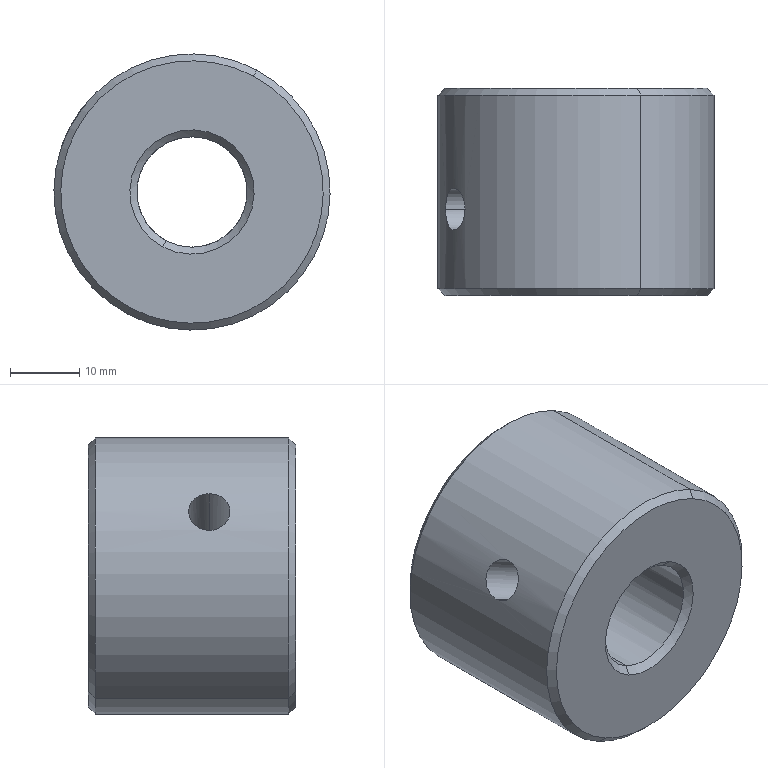Component | SolidWorks | TopMaterialTray-4 | 1 solid | 16 faces | box 40 x 30 x 40 mm | volume 31150 mm3 | cone 8 | cylinder 6 | plane 2 | commonest cylinder face diameters 6 x2 40 x2 16 x2
STEP:
#1=CARTESIAN_POINT('',(5.47,-4.508,-5.24));
#2=VERTEX_POINT('',#1);
#3=CARTESIAN_POINT('',(5.359,-4.508,-5.449));
#4=VERTEX_POINT('',#3);
#5=CARTESIAN_POINT('',(5.47,-4.508,-5.24));
#6=CARTESIAN_POINT('',(5.47,-4.516,-5.24));
#7=CARTESIAN_POINT('',(5.469,-4.523,-5.241));
#8=CARTESIAN_POINT('',(5.467,-4.539,-5.243));
#9=CARTESIAN_POINT('',(5.466,-4.546,-5.245));
#10=CARTESIAN_POINT('',(5.463,-4.56,-5.25));
#11=CARTESIAN_POINT('',(5.46,-4.567,-5.253));
#12=CARTESIAN_POINT('',(5.455,-4.58,-5.26));
#13=CARTESIAN_POINT('',(5.453,-4.586,-5.264));
#14=CARTESIAN_POINT('',(5.446,-4.597,-5.273));
#15=CARTESIAN_POINT('',(5.443,-4.602,-5.278));
#16=CARTESIAN_POINT('',(5.436,-4.61,-5.289));
#17=CARTESIAN_POINT('',(5.433,-4.614,-5.295));
#18=CARTESIAN_POINT('',(5.425,-4.62,-5.307));
#19=CARTESIAN_POINT('',(5.421,-4.622,-5.313));
#20=CARTESIAN_POINT('',(5.414,-4.625,-5.326));
#21=CARTESIAN_POINT('',(5.41,-4.626,-5.333));
#22=CARTESIAN_POINT('',(5.403,-4.626,-5.347));
#23=CARTESIAN_POINT('',(5.399,-4.625,-5.354));
#24=CARTESIAN_POINT('',(5.393,-4.622,-5.367));
#25=CARTESIAN_POINT('',(5.389,-4.62,-5.374));
#26=CARTESIAN_POINT('',(5.384,-4.614,-5.387));
#27=CARTESIAN_POINT('',(5.381,-4.61,-5.393));
#28=CARTESIAN_POINT('',(5.376,-4.602,-5.405));
#29=CARTESIAN_POINT('',(5.373,-4.597,-5.411));
#30=CARTESIAN_POINT('',(5.369,-4.586,-5.421));
#31=CARTESIAN_POINT('',(5.368,-4.58,-5.426));
#32=CARTESIAN_POINT('',(5.364,-4.567,-5.434));
#33=CARTESIAN_POINT('',(5.363,-4.56,-5.437));
#34=CARTESIAN_POINT('',(5.361,-4.546,-5.443));
#35=CARTESIAN_POINT('',(5.36,-4.539,-5.445));
#36=CARTESIAN_POINT('',(5.359,-4.523,-5.448));
#37=CARTESIAN_POINT('',(5.359,-4.516,-5.449));
#38=CARTESIAN_POINT('',(5.359,-4.508,-5.449));
#39=B_SPLINE_CURVE_WITH_KNOTS('',3,(#5,#6,#7,#8,#9,#10,#11,#12,#13,#14,#15,#16,#17,#18,#19,#20,#21,#22,#23,#24,#25,#26,#27,#28,#29,#30,#31,#32,#33,#34,#35,#36,#37,#38),.UNSPECIFIED.,.F.,.F.,(4,2,2,2,2,2,2,2,2,2,2,2,2,2,2,2,4),(0.009393,0.00998,0.01057,0.01115,0.01174,0.01233,0.01291,0.0135,0.01409,0.01467,0.01526,0.01585,0.01644,0.01702,0.01761,0.0182,0.01878),.UNSPECIFIED.);
#40=EDGE_CURVE('',#2,#4,#39,.T.);
#41=ORIENTED_EDGE('',*,*,#40,.F.);
#42=CARTESIAN_POINT('',(5.9,-4.508,-5.468));
#43=VERTEX_POINT('',#42);
#44=CARTESIAN_POINT('',(6.018,-4.508,-5.531));
#45=DIRECTION('',(0.8837,-0.,-0.468));
#46=VECTOR('',#45,39.37);
#47=LINE('',#44,#46);
#48=EDGE_CURVE('',#2,#43,#47,.T.);
#49=ORIENTED_EDGE('',*,*,#48,.T.);
#50=CARTESIAN_POINT('',(5.789,-4.508,-5.676));
#51=VERTEX_POINT('',#50);
#52=CARTESIAN_POINT('',(5.9,-4.508,-5.468));
#53=CARTESIAN_POINT('',(5.9,-4.516,-5.468));
#54=CARTESIAN_POINT('',(5.899,-4.523,-5.468));
#55=CARTESIAN_POINT('',(5.896,-4.539,-5.47));
#56=CARTESIAN_POINT('',(5.895,-4.546,-5.472));
#57=CARTESIAN_POINT('',(5.89,-4.56,-5.476));
#58=CARTESIAN_POINT('',(5.887,-4.567,-5.479));
#59=CARTESIAN_POINT('',(5.881,-4.58,-5.485));
#60=CARTESIAN_POINT('',(5.877,-4.586,-5.489));
#61=CARTESIAN_POINT('',(5.869,-4.597,-5.497));
#62=CARTESIAN_POINT('',(5.865,-4.602,-5.501));
#63=CARTESIAN_POINT('',(5.857,-4.61,-5.511));
#64=CARTESIAN_POINT('',(5.852,-4.614,-5.517));
#65=CARTESIAN_POINT('',(5.844,-4.62,-5.529));
#66=CARTESIAN_POINT('',(5.84,-4.622,-5.535));
#67=CARTESIAN_POINT('',(5.832,-4.625,-5.548));
#68=CARTESIAN_POINT('',(5.828,-4.626,-5.554));
#69=CARTESIAN_POINT('',(5.82,-4.626,-5.568));
#70=CARTESIAN_POINT('',(5.817,-4.625,-5.575));
#71=CARTESIAN_POINT('',(5.811,-4.622,-5.589));
#72=CARTESIAN_POINT('',(5.808,-4.62,-5.596));
#73=CARTESIAN_POINT('',(5.803,-4.614,-5.61));
#74=CARTESIAN_POINT('',(5.801,-4.61,-5.616));
#75=CARTESIAN_POINT('',(5.798,-4.602,-5.629));
#76=CARTESIAN_POINT('',(5.796,-4.597,-5.635));
#77=CARTESIAN_POINT('',(5.794,-4.586,-5.646));
#78=CARTESIAN_POINT('',(5.793,-4.58,-5.651));
#79=CARTESIAN_POINT('',(5.791,-4.567,-5.66));
#80=CARTESIAN_POINT('',(5.791,-4.56,-5.664));
#81=CARTESIAN_POINT('',(5.79,-4.546,-5.67));
#82=CARTESIAN_POINT('',(5.79,-4.539,-5.672));
#83=CARTESIAN_POINT('',(5.789,-4.523,-5.676));
#84=CARTESIAN_POINT('',(5.789,-4.516,-5.676));
#85=CARTESIAN_POINT('',(5.789,-4.508,-5.676));
#86=B_SPLINE_CURVE_WITH_KNOTS('',3,(#52,#53,#54,#55,#56,#57,#58,#59,#60,#61,#62,#63,#64,#65,#66,#67,#68,#69,#70,#71,#72,#73,#74,#75,#76,#77,#78,#79,#80,#81,#82,#83,#84,#85),.UNSPECIFIED.,.F.,.F.,(4,2,2,2,2,2,2,2,2,2,2,2,2,2,2,2,4),(0.009466,0.01006,0.01065,0.01124,0.01183,0.01242,0.01302,0.01361,0.0142,0.01479,0.01538,0.01597,0.01656,0.01716,0.01775,0.01834,0.01893),.UNSPECIFIED.);
#87=EDGE_CURVE('',#43,#51,#86,.T.);
#88=ORIENTED_EDGE('',*,*,#87,.T.);
#89=CARTESIAN_POINT('',(5.908,-4.508,-5.739));
#90=DIRECTION('',(0.8837,-0.,-0.468));
#91=VECTOR('',#90,39.37);
#92=LINE('',#89,#91);
#93=EDGE_CURVE('',#4,#51,#92,.T.);
#94=ORIENTED_EDGE('',*,*,#93,.F.);
#95=EDGE_LOOP('',(#41,#49,#88,#94));
#96=FACE_OUTER_BOUND('',#95,.T.);
#97=CARTESIAN_POINT('',(5.963,-4.508,-5.635));
#98=DIRECTION('',(0.8837,-0.,-0.468));
#99=DIRECTION('',(-0.468,0.,-0.8837));
#100=AXIS2_PLACEMENT_3D('',#97,#98,#99);
#101=CYLINDRICAL_SURFACE('',#100,0.1181);
#102=ADVANCED_FACE('',(#96),#101,.F.);
#103=CARTESIAN_POINT('',(5.752,-5.,-6.37));
#104=VERTEX_POINT('',#103);
#105=CARTESIAN_POINT('',(6.452,-5.,-5.048));
#106=VERTEX_POINT('',#105);
#107=CARTESIAN_POINT('',(6.102,-5.,-5.709));
#108=DIRECTION('',(0.,1.,0.));
#109=DIRECTION('',(-0.468,0.,-0.8837));
#110=AXIS2_PLACEMENT_3D('',#107,#108,#109);
#111=CIRCLE('',#110,0.748);
#112=EDGE_CURVE('',#104,#106,#111,.T.);
#113=ORIENTED_EDGE('',*,*,#112,.T.);
#114=CARTESIAN_POINT('',(6.471,-4.961,-5.013));
#115=VERTEX_POINT('',#114);
#116=CARTESIAN_POINT('',(6.471,-4.961,-5.013));
#117=DIRECTION('',(0.3309,0.7071,0.6249));
#118=VECTOR('',#117,39.37);
#119=LINE('',#116,#118);
#120=EDGE_CURVE('',#106,#115,#119,.T.);
#121=ORIENTED_EDGE('',*,*,#120,.T.);
#122=CARTESIAN_POINT('',(5.734,-4.961,-6.405));
#123=VERTEX_POINT('',#122);
#124=CARTESIAN_POINT('',(6.102,-4.961,-5.709));
#125=DIRECTION('',(0.,1.,0.));
#126=DIRECTION('',(0.468,-0.,0.8837));
#127=AXIS2_PLACEMENT_3D('',#124,#125,#126);
#128=CIRCLE('',#127,0.7874);
#129=EDGE_CURVE('',#123,#115,#128,.T.);
#130=ORIENTED_EDGE('',*,*,#129,.F.);
#131=CARTESIAN_POINT('',(5.734,-4.961,-6.405));
#132=DIRECTION('',(-0.3309,0.7071,-0.6249));
#133=VECTOR('',#132,39.37);
#134=LINE('',#131,#133);
#135=EDGE_CURVE('',#104,#123,#134,.T.);
#136=ORIENTED_EDGE('',*,*,#135,.F.);
#137=EDGE_LOOP('',(#113,#121,#130,#136));
#138=FACE_OUTER_BOUND('',#137,.T.);
#139=CARTESIAN_POINT('',(6.102,-4.961,-5.709));
#140=DIRECTION('',(0.,1.,0.));
#141=DIRECTION('',(-0.468,0.,-0.8837));
#142=AXIS2_PLACEMENT_3D('',#139,#140,#141);
#143=CONICAL_SURFACE('',#142,0.7874,0.7854);
#144=ADVANCED_FACE('',(#138),#143,.T.);
#145=CARTESIAN_POINT('',(6.452,-3.819,-5.048));
#146=VERTEX_POINT('',#145);
#147=CARTESIAN_POINT('',(5.752,-3.819,-6.37));
#148=VERTEX_POINT('',#147);
#149=CARTESIAN_POINT('',(6.102,-3.819,-5.709));
#150=DIRECTION('',(-0.,-1.,-0.));
#151=DIRECTION('',(0.468,-0.,0.8837));
#152=AXIS2_PLACEMENT_3D('',#149,#150,#151);
#153=CIRCLE('',#152,0.748);
#154=EDGE_CURVE('',#146,#148,#153,.T.);
#155=ORIENTED_EDGE('',*,*,#154,.T.);
#156=CARTESIAN_POINT('',(5.734,-3.858,-6.405));
#157=VERTEX_POINT('',#156);
#158=CARTESIAN_POINT('',(5.734,-3.858,-6.405));
#159=DIRECTION('',(-0.3309,-0.7071,-0.6249));
#160=VECTOR('',#159,39.37);
#161=LINE('',#158,#160);
#162=EDGE_CURVE('',#148,#157,#161,.T.);
#163=ORIENTED_EDGE('',*,*,#162,.T.);
#164=CARTESIAN_POINT('',(6.471,-3.858,-5.013));
#165=VERTEX_POINT('',#164);
#166=CARTESIAN_POINT('',(6.102,-3.858,-5.709));
#167=DIRECTION('',(-0.,-1.,-0.));
#168=DIRECTION('',(0.468,-0.,0.8837));
#169=AXIS2_PLACEMENT_3D('',#166,#167,#168);
#170=CIRCLE('',#169,0.7874);
#171=EDGE_CURVE('',#165,#157,#170,.T.);
#172=ORIENTED_EDGE('',*,*,#171,.F.);
#173=CARTESIAN_POINT('',(6.471,-3.858,-5.013));
#174=DIRECTION('',(0.3309,-0.7071,0.6249));
#175=VECTOR('',#174,39.37);
#176=LINE('',#173,#175);
#177=EDGE_CURVE('',#146,#165,#176,.T.);
#178=ORIENTED_EDGE('',*,*,#177,.F.);
#179=EDGE_LOOP('',(#155,#163,#172,#178));
#180=FACE_OUTER_BOUND('',#179,.T.);
#181=CARTESIAN_POINT('',(6.102,-3.858,-5.709));
#182=DIRECTION('',(-0.,-1.,-0.));
#183=DIRECTION('',(0.468,-0.,0.8837));
#184=AXIS2_PLACEMENT_3D('',#181,#182,#183);
#185=CONICAL_SURFACE('',#184,0.7874,0.7854);
#186=ADVANCED_FACE('',(#180),#185,.T.);
#187=CARTESIAN_POINT('',(5.955,-4.961,-5.987));
#188=VERTEX_POINT('',#187);
#189=CARTESIAN_POINT('',(6.25,-4.961,-5.43));
#190=VERTEX_POINT('',#189);
#191=CARTESIAN_POINT('',(6.102,-4.961,-5.709));
#192=DIRECTION('',(-0.,-1.,-0.));
#193=DIRECTION('',(0.468,0.,0.8837));
#194=AXIS2_PLACEMENT_3D('',#191,#192,#193);
#195=CIRCLE('',#194,0.315);
#196=EDGE_CURVE('',#188,#190,#195,.T.);
#197=ORIENTED_EDGE('',*,*,#196,.F.);
#198=CARTESIAN_POINT('',(5.937,-5.,-6.022));
#199=VERTEX_POINT('',#198);
#200=CARTESIAN_POINT('',(5.937,-5.,-6.022));
#201=DIRECTION('',(-0.3309,-0.7071,-0.6249));
#202=VECTOR('',#201,39.37);
#203=LINE('',#200,#202);
#204=EDGE_CURVE('',#188,#199,#203,.T.);
#205=ORIENTED_EDGE('',*,*,#204,.T.);
#206=CARTESIAN_POINT('',(6.268,-5.,-5.396));
#207=VERTEX_POINT('',#206);
#208=CARTESIAN_POINT('',(6.102,-5.,-5.709));
#209=DIRECTION('',(0.,1.,0.));
#210=DIRECTION('',(0.468,-0.,0.8837));
#211=AXIS2_PLACEMENT_3D('',#208,#209,#210);
#212=CIRCLE('',#211,0.3543);
#213=EDGE_CURVE('',#207,#199,#212,.T.);
#214=ORIENTED_EDGE('',*,*,#213,.F.);
#215=CARTESIAN_POINT('',(6.268,-5.,-5.396));
#216=DIRECTION('',(0.3309,-0.7071,0.6249));
#217=VECTOR('',#216,39.37);
#218=LINE('',#215,#217);
#219=EDGE_CURVE('',#190,#207,#218,.T.);
#220=ORIENTED_EDGE('',*,*,#219,.F.);
#221=EDGE_LOOP('',(#197,#205,#214,#220));
#222=FACE_OUTER_BOUND('',#221,.T.);
#223=CARTESIAN_POINT('',(6.102,-5.,-5.709));
#224=DIRECTION('',(-0.,-1.,-0.));
#225=DIRECTION('',(0.468,-0.,0.8837));
#226=AXIS2_PLACEMENT_3D('',#223,#224,#225);
#227=CONICAL_SURFACE('',#226,0.3543,0.7854);
#228=ADVANCED_FACE('',(#222),#227,.F.);
#229=CARTESIAN_POINT('',(6.25,-3.858,-5.43));
#230=VERTEX_POINT('',#229);
#231=CARTESIAN_POINT('',(5.824,-3.858,-5.561));
#232=VERTEX_POINT('',#231);
#233=CARTESIAN_POINT('',(6.102,-3.858,-5.709));
#234=DIRECTION('',(-0.,-1.,-0.));
#235=DIRECTION('',(-0.468,0.,-0.8837));
#236=AXIS2_PLACEMENT_3D('',#233,#234,#235);
#237=CIRCLE('',#236,0.315);
#238=EDGE_CURVE('',#230,#232,#237,.T.);
#239=ORIENTED_EDGE('',*,*,#238,.T.);
#240=CARTESIAN_POINT('',(5.789,-3.819,-5.543));
#241=VERTEX_POINT('',#240);
#242=CARTESIAN_POINT('',(5.789,-3.819,-5.543));
#243=DIRECTION('',(-0.6249,0.7071,0.3309));
#244=VECTOR('',#243,39.37);
#245=LINE('',#242,#244);
#246=EDGE_CURVE('',#232,#241,#245,.T.);
#247=ORIENTED_EDGE('',*,*,#246,.T.);
#248=CARTESIAN_POINT('',(6.415,-3.819,-5.874));
#249=VERTEX_POINT('',#248);
#250=CARTESIAN_POINT('',(6.102,-3.819,-5.709));
#251=DIRECTION('',(-0.,-1.,-0.));
#252=DIRECTION('',(0.8837,0.,-0.468));
#253=AXIS2_PLACEMENT_3D('',#250,#251,#252);
#254=CIRCLE('',#253,0.3543);
#255=EDGE_CURVE('',#249,#241,#254,.T.);
#256=ORIENTED_EDGE('',*,*,#255,.F.);
#257=CARTESIAN_POINT('',(6.381,-3.858,-5.856));
#258=VERTEX_POINT('',#257);
#259=CARTESIAN_POINT('',(6.415,-3.819,-5.874));
#260=DIRECTION('',(0.6249,0.7071,-0.3309));
#261=VECTOR('',#260,39.37);
#262=LINE('',#259,#261);
#263=EDGE_CURVE('',#258,#249,#262,.T.);
#264=ORIENTED_EDGE('',*,*,#263,.F.);
#265=CARTESIAN_POINT('',(6.102,-3.858,-5.709));
#266=DIRECTION('',(-0.,-1.,-0.));
#267=DIRECTION('',(-0.468,0.,-0.8837));
#268=AXIS2_PLACEMENT_3D('',#265,#266,#267);
#269=CIRCLE('',#268,0.315);
#270=EDGE_CURVE('',#258,#230,#269,.T.);
#271=ORIENTED_EDGE('',*,*,#270,.T.);
#272=EDGE_LOOP('',(#239,#247,#256,#264,#271));
#273=FACE_OUTER_BOUND('',#272,.T.);
#274=CARTESIAN_POINT('',(6.102,-3.819,-5.709));
#275=DIRECTION('',(0.,1.,0.));
#276=DIRECTION('',(0.8837,0.,-0.468));
#277=AXIS2_PLACEMENT_3D('',#274,#275,#276);
#278=CONICAL_SURFACE('',#277,0.3543,0.7854);
#279=ADVANCED_FACE('',(#273),#278,.F.);
#280=CARTESIAN_POINT('',(5.359,-4.508,-5.449));
#281=CARTESIAN_POINT('',(5.359,-4.5,-5.449));
#282=CARTESIAN_POINT('',(5.359,-4.492,-5.448));
#283=CARTESIAN_POINT('',(5.36,-4.477,-5.445));
#284=CARTESIAN_POINT('',(5.361,-4.47,-5.443));
#285=CARTESIAN_POINT('',(5.363,-4.455,-5.437));
#286=CARTESIAN_POINT('',(5.364,-4.449,-5.434));
#287=CARTESIAN_POINT('',(5.368,-4.436,-5.426));
#288=CARTESIAN_POINT('',(5.369,-4.43,-5.421));
#289=CARTESIAN_POINT('',(5.373,-4.419,-5.411));
#290=CARTESIAN_POINT('',(5.376,-4.414,-5.405));
#291=CARTESIAN_POINT('',(5.381,-4.405,-5.394));
#292=CARTESIAN_POINT('',(5.384,-4.402,-5.387));
#293=CARTESIAN_POINT('',(5.389,-4.396,-5.374));
#294=CARTESIAN_POINT('',(5.393,-4.394,-5.368));
#295=CARTESIAN_POINT('',(5.399,-4.391,-5.354));
#296=CARTESIAN_POINT('',(5.403,-4.39,-5.347));
#297=CARTESIAN_POINT('',(5.41,-4.39,-5.333));
#298=CARTESIAN_POINT('',(5.414,-4.391,-5.327));
#299=CARTESIAN_POINT('',(5.421,-4.394,-5.313));
#300=CARTESIAN_POINT('',(5.425,-4.396,-5.307));
#301=CARTESIAN_POINT('',(5.433,-4.402,-5.295));
#302=CARTESIAN_POINT('',(5.436,-4.405,-5.289));
#303=CARTESIAN_POINT('',(5.443,-4.414,-5.278));
#304=CARTESIAN_POINT('',(5.446,-4.419,-5.273));
#305=CARTESIAN_POINT('',(5.453,-4.43,-5.264));
#306=CARTESIAN_POINT('',(5.455,-4.436,-5.26));
#307=CARTESIAN_POINT('',(5.46,-4.449,-5.253));
#308=CARTESIAN_POINT('',(5.463,-4.456,-5.25));
#309=CARTESIAN_POINT('',(5.466,-4.47,-5.245));
#310=CARTESIAN_POINT('',(5.467,-4.477,-5.243));
#311=CARTESIAN_POINT('',(5.469,-4.492,-5.241));
#312=CARTESIAN_POINT('',(5.47,-4.5,-5.24));
#313=CARTESIAN_POINT('',(5.47,-4.508,-5.24));
#314=B_SPLINE_CURVE_WITH_KNOTS('',3,(#280,#281,#282,#283,#284,#285,#286,#287,#288,#289,#290,#291,#292,#293,#294,#295,#296,#297,#298,#299,#300,#301,#302,#303,#304,#305,#306,#307,#308,#309,#310,#311,#312,#313),.UNSPECIFIED.,.F.,.F.,(4,2,2,2,2,2,2,2,2,2,2,2,2,2,2,2,4),(0.,0.000587,0.001174,0.001761,0.002348,0.002935,0.003522,0.004109,0.004696,0.005283,0.00587,0.006457,0.007044,0.007631,0.008219,0.008806,0.009393),.UNSPECIFIED.);
#315=EDGE_CURVE('',#4,#2,#314,.T.);
#316=ORIENTED_EDGE('',*,*,#315,.T.);
#317=ORIENTED_EDGE('',*,*,#40,.T.);
#318=EDGE_LOOP('',(#316,#317));
#319=FACE_BOUND('',#318,.T.);
#320=ORIENTED_EDGE('',*,*,#171,.T.);
#321=CARTESIAN_POINT('',(5.734,-5.,-6.405));
#322=DIRECTION('',(-0.,-1.,-0.));
#323=VECTOR('',#322,39.37);
#324=LINE('',#321,#323);
#325=EDGE_CURVE('',#157,#123,#324,.T.);
#326=ORIENTED_EDGE('',*,*,#325,.T.);
#327=ORIENTED_EDGE('',*,*,#129,.T.);
#328=CARTESIAN_POINT('',(6.471,-5.,-5.013));
#329=DIRECTION('',(-0.,-1.,-0.));
#330=VECTOR('',#329,39.37);
#331=LINE('',#328,#330);
#332=EDGE_CURVE('',#165,#115,#331,.T.);
#333=ORIENTED_EDGE('',*,*,#332,.F.);
#334=EDGE_LOOP('',(#320,#326,#327,#333));
#335=FACE_OUTER_BOUND('',#334,.T.);
#336=CARTESIAN_POINT('',(6.102,-5.,-5.709));
#337=DIRECTION('',(-0.,-1.,-0.));
#338=DIRECTION('',(0.468,-0.,0.8837));
#339=AXIS2_PLACEMENT_3D('',#336,#337,#338);
#340=CYLINDRICAL_SURFACE('',#339,0.7874);
#341=ADVANCED_FACE('',(#319,#335),#340,.T.);
#342=ORIENTED_EDGE('',*,*,#196,.T.);
#343=CARTESIAN_POINT('',(6.25,-5.,-5.43));
#344=DIRECTION('',(0.,1.,0.));
#345=VECTOR('',#344,39.37);
#346=LINE('',#343,#345);
#347=EDGE_CURVE('',#190,#230,#346,.T.);
#348=ORIENTED_EDGE('',*,*,#347,.T.);
#349=ORIENTED_EDGE('',*,*,#270,.F.);
#350=CARTESIAN_POINT('',(5.955,-3.858,-5.987));
#351=VERTEX_POINT('',#350);
#352=CARTESIAN_POINT('',(6.102,-3.858,-5.709));
#353=DIRECTION('',(-0.,-1.,-0.));
#354=DIRECTION('',(-0.468,0.,-0.8837));
#355=AXIS2_PLACEMENT_3D('',#352,#353,#354);
#356=CIRCLE('',#355,0.315);
#357=EDGE_CURVE('',#351,#258,#356,.T.);
#358=ORIENTED_EDGE('',*,*,#357,.F.);
#359=CARTESIAN_POINT('',(5.955,-5.,-5.987));
#360=DIRECTION('',(0.,1.,0.));
#361=VECTOR('',#360,39.37);
#362=LINE('',#359,#361);
#363=EDGE_CURVE('',#188,#351,#362,.T.);
#364=ORIENTED_EDGE('',*,*,#363,.F.);
#365=EDGE_LOOP('',(#342,#348,#349,#358,#364));
#366=FACE_OUTER_BOUND('',#365,.T.);
#367=CARTESIAN_POINT('',(6.102,-5.,-5.709));
#368=DIRECTION('',(0.,1.,0.));
#369=DIRECTION('',(-0.468,0.,-0.8837));
#370=AXIS2_PLACEMENT_3D('',#367,#368,#369);
#371=CYLINDRICAL_SURFACE('',#370,0.315);
#372=ADVANCED_FACE('',(#366),#371,.F.);
#373=ORIENTED_EDGE('',*,*,#347,.F.);
#374=CARTESIAN_POINT('',(6.102,-4.961,-5.709));
#375=DIRECTION('',(-0.,-1.,-0.));
#376=DIRECTION('',(0.468,0.,0.8837));
#377=AXIS2_PLACEMENT_3D('',#374,#375,#376);
#378=CIRCLE('',#377,0.315);
#379=EDGE_CURVE('',#190,#188,#378,.T.);
#380=ORIENTED_EDGE('',*,*,#379,.T.);
#381=ORIENTED_EDGE('',*,*,#363,.T.);
#382=CARTESIAN_POINT('',(6.102,-3.858,-5.709));
#383=DIRECTION('',(-0.,-1.,-0.));
#384=DIRECTION('',(-0.468,0.,-0.8837));
#385=AXIS2_PLACEMENT_3D('',#382,#383,#384);
#386=CIRCLE('',#385,0.315);
#387=EDGE_CURVE('',#232,#351,#386,.T.);
#388=ORIENTED_EDGE('',*,*,#387,.F.);
#389=ORIENTED_EDGE('',*,*,#238,.F.);
#390=EDGE_LOOP('',(#373,#380,#381,#388,#389));
#391=FACE_OUTER_BOUND('',#390,.T.);
#392=CARTESIAN_POINT('',(5.789,-4.508,-5.676));
#393=CARTESIAN_POINT('',(5.789,-4.5,-5.676));
#394=CARTESIAN_POINT('',(5.789,-4.492,-5.676));
#395=CARTESIAN_POINT('',(5.79,-4.477,-5.672));
#396=CARTESIAN_POINT('',(5.79,-4.47,-5.67));
#397=CARTESIAN_POINT('',(5.791,-4.455,-5.664));
#398=CARTESIAN_POINT('',(5.791,-4.449,-5.66));
#399=CARTESIAN_POINT('',(5.793,-4.436,-5.651));
#400=CARTESIAN_POINT('',(5.794,-4.43,-5.646));
#401=CARTESIAN_POINT('',(5.797,-4.414,-5.629));
#402=CARTESIAN_POINT('',(5.801,-4.405,-5.617));
#403=CARTESIAN_POINT('',(5.808,-4.396,-5.596));
#404=CARTESIAN_POINT('',(5.811,-4.394,-5.589));
#405=CARTESIAN_POINT('',(5.817,-4.391,-5.575));
#406=CARTESIAN_POINT('',(5.82,-4.39,-5.568));
#407=CARTESIAN_POINT('',(5.828,-4.39,-5.554));
#408=CARTESIAN_POINT('',(5.832,-4.391,-5.548));
#409=CARTESIAN_POINT('',(5.84,-4.394,-5.535));
#410=CARTESIAN_POINT('',(5.844,-4.396,-5.529));
#411=CARTESIAN_POINT('',(5.853,-4.402,-5.517));
#412=CARTESIAN_POINT('',(5.857,-4.406,-5.511));
#413=CARTESIAN_POINT('',(5.865,-4.414,-5.501));
#414=CARTESIAN_POINT('',(5.869,-4.419,-5.497));
#415=CARTESIAN_POINT('',(5.877,-4.43,-5.489));
#416=CARTESIAN_POINT('',(5.881,-4.436,-5.485));
#417=CARTESIAN_POINT('',(5.887,-4.448,-5.479));
#418=CARTESIAN_POINT('',(5.89,-4.455,-5.476));
#419=CARTESIAN_POINT('',(5.895,-4.47,-5.472));
#420=CARTESIAN_POINT('',(5.896,-4.477,-5.47));
#421=CARTESIAN_POINT('',(5.899,-4.492,-5.468));
#422=CARTESIAN_POINT('',(5.9,-4.5,-5.468));
#423=CARTESIAN_POINT('',(5.9,-4.508,-5.468));
#424=B_SPLINE_CURVE_WITH_KNOTS('',3,(#392,#393,#394,#395,#396,#397,#398,#399,#400,#401,#402,#403,#404,#405,#406,#407,#408,#409,#410,#411,#412,#413,#414,#415,#416,#417,#418,#419,#420,#421,#422,#423),.UNSPECIFIED.,.F.,.F.,(4,2,2,2,2,2,2,2,2,2,2,2,2,2,2,4),(0.,0.0005916,0.001183,0.001775,0.002367,0.00355,0.004142,0.004733,0.005325,0.005916,0.006508,0.0071,0.007691,0.008283,0.008875,0.009466),.UNSPECIFIED.);
#425=EDGE_CURVE('',#51,#43,#424,.T.);
#426=ORIENTED_EDGE('',*,*,#425,.F.);
#427=ORIENTED_EDGE('',*,*,#87,.F.);
#428=EDGE_LOOP('',(#426,#427));
#429=FACE_BOUND('',#428,.T.);
#430=CARTESIAN_POINT('',(6.102,-5.,-5.709));
#431=DIRECTION('',(0.,1.,0.));
#432=DIRECTION('',(-0.468,0.,-0.8837));
#433=AXIS2_PLACEMENT_3D('',#430,#431,#432);
#434=CYLINDRICAL_SURFACE('',#433,0.315);
#435=ADVANCED_FACE('',(#391,#429),#434,.F.);
#436=ORIENTED_EDGE('',*,*,#325,.F.);
#437=CARTESIAN_POINT('',(6.102,-3.858,-5.709));
#438=DIRECTION('',(-0.,-1.,-0.));
#439=DIRECTION('',(0.468,-0.,0.8837));
#440=AXIS2_PLACEMENT_3D('',#437,#438,#439);
#441=CIRCLE('',#440,0.7874);
#442=EDGE_CURVE('',#157,#165,#441,.T.);
#443=ORIENTED_EDGE('',*,*,#442,.T.);
#444=ORIENTED_EDGE('',*,*,#332,.T.);
#445=CARTESIAN_POINT('',(6.102,-4.961,-5.709));
#446=DIRECTION('',(0.,1.,0.));
#447=DIRECTION('',(0.468,-0.,0.8837));
#448=AXIS2_PLACEMENT_3D('',#445,#446,#447);
#449=CIRCLE('',#448,0.7874);
#450=EDGE_CURVE('',#115,#123,#449,.T.);
#451=ORIENTED_EDGE('',*,*,#450,.T.);
#452=EDGE_LOOP('',(#436,#443,#444,#451));
#453=FACE_OUTER_BOUND('',#452,.T.);
#454=CARTESIAN_POINT('',(6.102,-5.,-5.709));
#455=DIRECTION('',(-0.,-1.,-0.));
#456=DIRECTION('',(0.468,-0.,0.8837));
#457=AXIS2_PLACEMENT_3D('',#454,#455,#456);
#458=CYLINDRICAL_SURFACE('',#457,0.7874);
#459=ADVANCED_FACE('',(#453),#458,.T.);
#460=ORIENTED_EDGE('',*,*,#120,.F.);
#461=CARTESIAN_POINT('',(6.102,-5.,-5.709));
#462=DIRECTION('',(0.,1.,0.));
#463=DIRECTION('',(-0.468,0.,-0.8837));
#464=AXIS2_PLACEMENT_3D('',#461,#462,#463);
#465=CIRCLE('',#464,0.748);
#466=EDGE_CURVE('',#106,#104,#465,.T.);
#467=ORIENTED_EDGE('',*,*,#466,.T.);
#468=ORIENTED_EDGE('',*,*,#135,.T.);
#469=ORIENTED_EDGE('',*,*,#450,.F.);
#470=EDGE_LOOP('',(#460,#467,#468,#469));
#471=FACE_OUTER_BOUND('',#470,.T.);
#472=CARTESIAN_POINT('',(6.102,-4.961,-5.709));
#473=DIRECTION('',(0.,1.,0.));
#474=DIRECTION('',(-0.468,0.,-0.8837));
#475=AXIS2_PLACEMENT_3D('',#472,#473,#474);
#476=CONICAL_SURFACE('',#475,0.7874,0.7854);
#477=ADVANCED_FACE('',(#471),#476,.T.);
#478=ORIENTED_EDGE('',*,*,#162,.F.);
#479=CARTESIAN_POINT('',(6.102,-3.819,-5.709));
#480=DIRECTION('',(-0.,-1.,-0.));
#481=DIRECTION('',(0.468,-0.,0.8837));
#482=AXIS2_PLACEMENT_3D('',#479,#480,#481);
#483=CIRCLE('',#482,0.748);
#484=EDGE_CURVE('',#148,#146,#483,.T.);
#485=ORIENTED_EDGE('',*,*,#484,.T.);
#486=ORIENTED_EDGE('',*,*,#177,.T.);
#487=ORIENTED_EDGE('',*,*,#442,.F.);
#488=EDGE_LOOP('',(#478,#485,#486,#487));
#489=FACE_OUTER_BOUND('',#488,.T.);
#490=CARTESIAN_POINT('',(6.102,-3.858,-5.709));
#491=DIRECTION('',(-0.,-1.,-0.));
#492=DIRECTION('',(0.468,-0.,0.8837));
#493=AXIS2_PLACEMENT_3D('',#490,#491,#492);
#494=CONICAL_SURFACE('',#493,0.7874,0.7854);
#495=ADVANCED_FACE('',(#489),#494,.T.);
#496=ORIENTED_EDGE('',*,*,#112,.F.);
#497=ORIENTED_EDGE('',*,*,#466,.F.);
#498=EDGE_LOOP('',(#496,#497));
#499=FACE_OUTER_BOUND('',#498,.T.);
#500=ORIENTED_EDGE('',*,*,#213,.T.);
#501=CARTESIAN_POINT('',(6.102,-5.,-5.709));
#502=DIRECTION('',(0.,1.,0.));
#503=DIRECTION('',(0.468,-0.,0.8837));
#504=AXIS2_PLACEMENT_3D('',#501,#502,#503);
#505=CIRCLE('',#504,0.3543);
#506=EDGE_CURVE('',#199,#207,#505,.T.);
#507=ORIENTED_EDGE('',*,*,#506,.T.);
#508=EDGE_LOOP('',(#500,#507));
#509=FACE_BOUND('',#508,.T.);
#510=CARTESIAN_POINT('',(5.407,-5.,-5.34));
#511=DIRECTION('',(-0.,-1.,-0.));
#512=DIRECTION('',(0.468,-0.,0.8837));
#513=AXIS2_PLACEMENT_3D('',#510,#511,#512);
#514=PLANE('',#513);
#515=ADVANCED_FACE('',(#499,#509),#514,.T.);
#516=ORIENTED_EDGE('',*,*,#154,.F.);
#517=ORIENTED_EDGE('',*,*,#484,.F.);
#518=EDGE_LOOP('',(#516,#517));
#519=FACE_OUTER_BOUND('',#518,.T.);
#520=ORIENTED_EDGE('',*,*,#255,.T.);
#521=CARTESIAN_POINT('',(6.102,-3.819,-5.709));
#522=DIRECTION('',(-0.,-1.,-0.));
#523=DIRECTION('',(0.8837,0.,-0.468));
#524=AXIS2_PLACEMENT_3D('',#521,#522,#523);
#525=CIRCLE('',#524,0.3543);
#526=EDGE_CURVE('',#241,#249,#525,.T.);
#527=ORIENTED_EDGE('',*,*,#526,.T.);
#528=EDGE_LOOP('',(#520,#527));
#529=FACE_BOUND('',#528,.T.);
#530=CARTESIAN_POINT('',(6.102,-3.819,-5.709));
#531=DIRECTION('',(0.,1.,0.));
#532=DIRECTION('',(-0.468,0.,-0.8837));
#533=AXIS2_PLACEMENT_3D('',#530,#531,#532);
#534=PLANE('',#533);
#535=ADVANCED_FACE('',(#519,#529),#534,.T.);
#536=ORIENTED_EDGE('',*,*,#204,.F.);
#537=ORIENTED_EDGE('',*,*,#379,.F.);
#538=ORIENTED_EDGE('',*,*,#219,.T.);
#539=ORIENTED_EDGE('',*,*,#506,.F.);
#540=EDGE_LOOP('',(#536,#537,#538,#539));
#541=FACE_OUTER_BOUND('',#540,.T.);
#542=CARTESIAN_POINT('',(6.102,-5.,-5.709));
#543=DIRECTION('',(-0.,-1.,-0.));
#544=DIRECTION('',(0.468,-0.,0.8837));
#545=AXIS2_PLACEMENT_3D('',#542,#543,#544);
#546=CONICAL_SURFACE('',#545,0.3543,0.7854);
#547=ADVANCED_FACE('',(#541),#546,.F.);
#548=ORIENTED_EDGE('',*,*,#246,.F.);
#549=ORIENTED_EDGE('',*,*,#387,.T.);
#550=ORIENTED_EDGE('',*,*,#357,.T.);
#551=ORIENTED_EDGE('',*,*,#263,.T.);
#552=ORIENTED_EDGE('',*,*,#526,.F.);
#553=EDGE_LOOP('',(#548,#549,#550,#551,#552));
#554=FACE_OUTER_BOUND('',#553,.T.);
#555=CARTESIAN_POINT('',(6.102,-3.819,-5.709));
#556=DIRECTION('',(0.,1.,0.));
#557=DIRECTION('',(0.8837,0.,-0.468));
#558=AXIS2_PLACEMENT_3D('',#555,#556,#557);
#559=CONICAL_SURFACE('',#558,0.3543,0.7854);
#560=ADVANCED_FACE('',(#554),#559,.F.);
#561=ORIENTED_EDGE('',*,*,#48,.F.);
#562=ORIENTED_EDGE('',*,*,#315,.F.);
#563=ORIENTED_EDGE('',*,*,#93,.T.);
#564=ORIENTED_EDGE('',*,*,#425,.T.);
#565=EDGE_LOOP('',(#561,#562,#563,#564));
#566=FACE_OUTER_BOUND('',#565,.T.);
#567=CARTESIAN_POINT('',(5.963,-4.508,-5.635));
#568=DIRECTION('',(0.8837,-0.,-0.468));
#569=DIRECTION('',(-0.468,0.,-0.8837));
#570=AXIS2_PLACEMENT_3D('',#567,#568,#569);
#571=CYLINDRICAL_SURFACE('',#570,0.1181);
#572=ADVANCED_FACE('',(#566),#571,.F.);
#573=CLOSED_SHELL('',(#102,#144,#186,#228,#279,#341,#372,#435,#459,#477,#495,#515,#535,#547,#560,#572));
#574=MANIFOLD_SOLID_BREP('',#573);
#575=CARTESIAN_POINT('',(0.,0.,0.));
#576=DIRECTION('',(0.,0.,1.));
#577=DIRECTION('',(1.,0.,0.));
#578=AXIS2_PLACEMENT_3D('',#575,#576,#577);
#579=(LENGTH_UNIT()NAMED_UNIT(*)SI_UNIT($,.METRE.));
#580=LENGTH_MEASURE_WITH_UNIT(LENGTH_MEASURE(0.0254),#579);
#581=DIMENSIONAL_EXPONENTS(1.,0.,0.,0.,0.,0.,0.);
#582=(CONVERSION_BASED_UNIT('',#580)LENGTH_UNIT()NAMED_UNIT(#581));
#583=UNCERTAINTY_MEASURE_WITH_UNIT(LENGTH_MEASURE(0.00001),#582,'','');
#584=(NAMED_UNIT(*)PLANE_ANGLE_UNIT()SI_UNIT($,.RADIAN.));
#585=(NAMED_UNIT(*)SI_UNIT($,.STERADIAN.)SOLID_ANGLE_UNIT());
#586=(GEOMETRIC_REPRESENTATION_CONTEXT(3)GLOBAL_UNCERTAINTY_ASSIGNED_CONTEXT((#583))GLOBAL_UNIT_ASSIGNED_CONTEXT((#582,#584,#585))REPRESENTATION_CONTEXT('',''));
#587=ADVANCED_BREP_SHAPE_REPRESENTATION('',(#574,#578),#586);
#588=COLOUR_RGB('',0.7922,0.8196,0.9333);
#589=FILL_AREA_STYLE_COLOUR('',#588);
#590=FILL_AREA_STYLE('',(#589));
#591=SURFACE_STYLE_FILL_AREA(#590);
#592=SURFACE_SIDE_STYLE('',(#591));
#593=SURFACE_STYLE_USAGE(.BOTH.,#592);
#594=PRESENTATION_STYLE_ASSIGNMENT((#593));
#595=STYLED_ITEM('',(#594),#574);
#596=(LENGTH_UNIT()NAMED_UNIT(*)SI_UNIT($,.METRE.));
#597=LENGTH_MEASURE_WITH_UNIT(LENGTH_MEASURE(0.0254),#596);
#598=DIMENSIONAL_EXPONENTS(1.,0.,0.,0.,0.,0.,0.);
#599=(CONVERSION_BASED_UNIT('',#597)LENGTH_UNIT()NAMED_UNIT(#598));
#600=UNCERTAINTY_MEASURE_WITH_UNIT(LENGTH_MEASURE(0.00001),#599,'','');
#601=(NAMED_UNIT(*)PLANE_ANGLE_UNIT()SI_UNIT($,.RADIAN.));
#602=(NAMED_UNIT(*)SI_UNIT($,.STERADIAN.)SOLID_ANGLE_UNIT());
#603=(GEOMETRIC_REPRESENTATION_CONTEXT(3)GLOBAL_UNCERTAINTY_ASSIGNED_CONTEXT((#600))GLOBAL_UNIT_ASSIGNED_CONTEXT((#599,#601,#602))REPRESENTATION_CONTEXT('',''));
#604=MECHANICAL_DESIGN_GEOMETRIC_PRESENTATION_REPRESENTATION('',(#595),#603);
#605=PRESENTATION_LAYER_ASSIGNMENT('','',(#595));